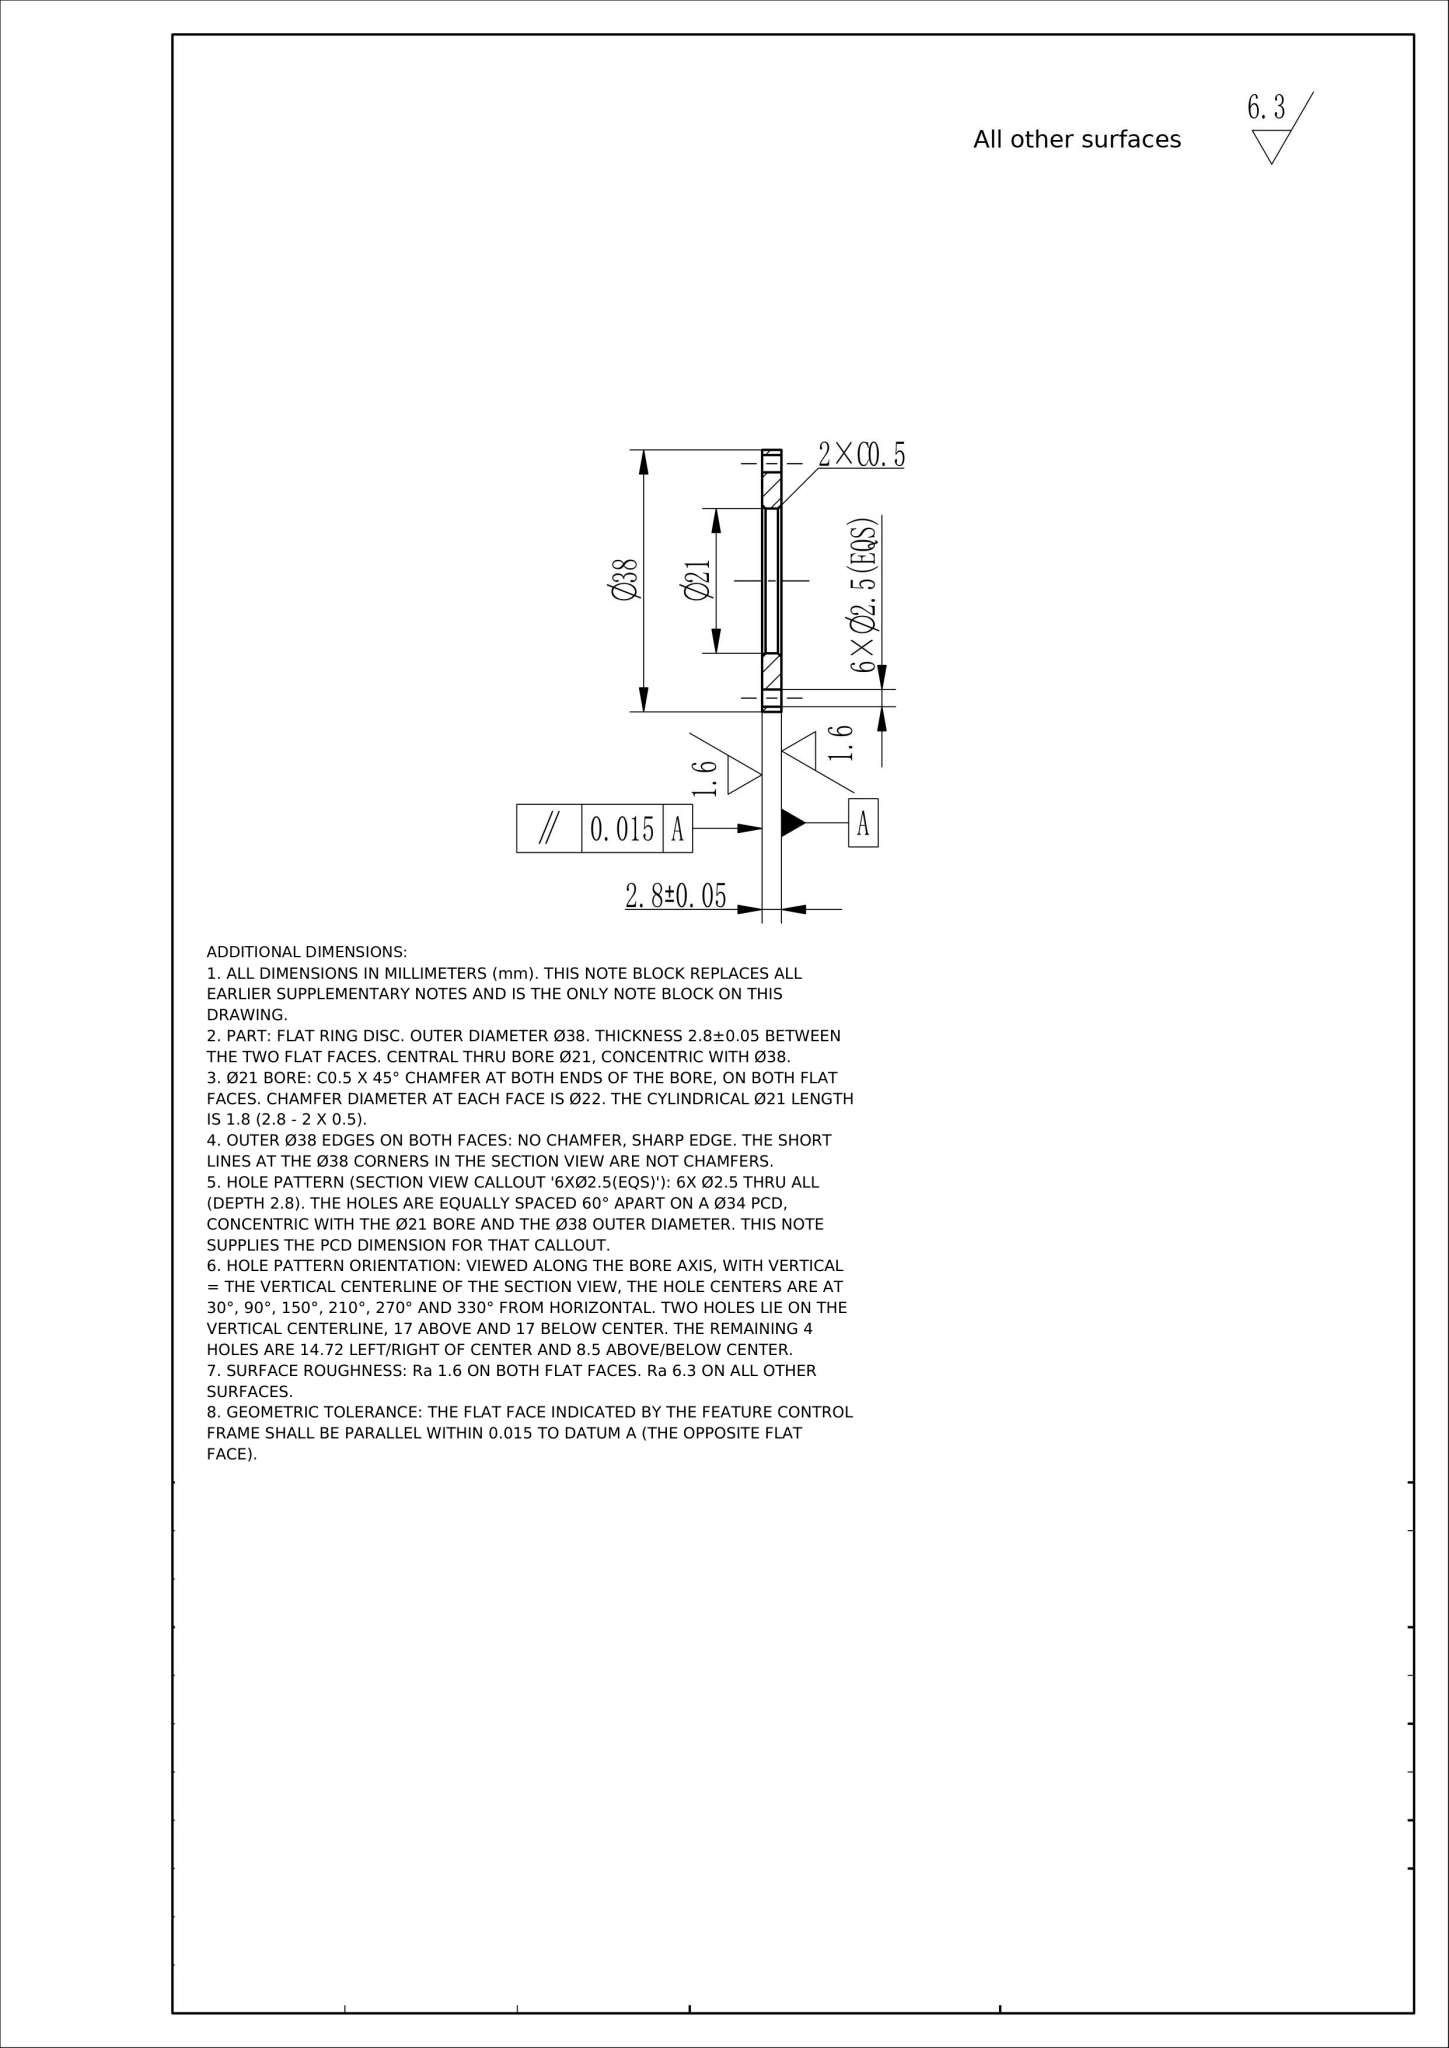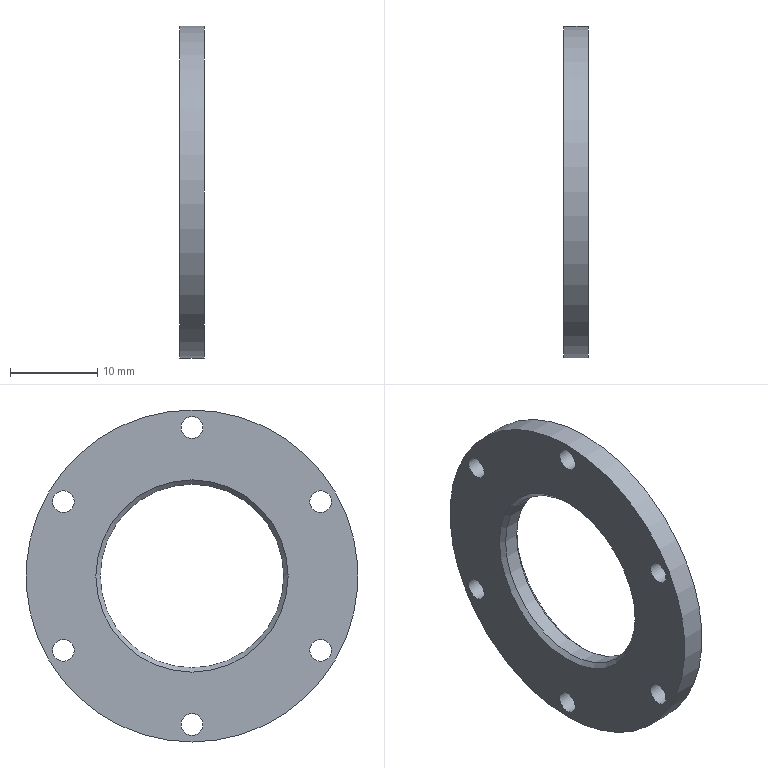Part | NX | mm | 1 solid | 12 faces | box 2.8 x 38 x 38 mm | volume 2106 mm3 | cylinder 8 | plane 2 | cone 2 | commonest cylinder face diameters 2.5 x6 38 x1 21 x1
STEP:
#1=CARTESIAN_POINT('',(0.,0.,0.));
#2=DIRECTION('',(0.,0.,1.));
#3=DIRECTION('',(1.,0.,0.));
#4=AXIS2_PLACEMENT_3D('',#1,#2,#3);
#5=(LENGTH_UNIT()NAMED_UNIT(*)SI_UNIT(.MILLI.,.METRE.));
#6=UNCERTAINTY_MEASURE_WITH_UNIT(LENGTH_MEASURE(0.00002),#5,'','');
#7=(NAMED_UNIT(*)PLANE_ANGLE_UNIT()SI_UNIT($,.RADIAN.));
#8=PLANE_ANGLE_MEASURE_WITH_UNIT(PLANE_ANGLE_MEASURE(0.01745),#7);
#9=DIMENSIONAL_EXPONENTS(0.,0.,0.,0.,0.,0.,0.);
#10=(CONVERSION_BASED_UNIT('',#8)NAMED_UNIT(#9)PLANE_ANGLE_UNIT());
#11=(NAMED_UNIT(*)SI_UNIT($,.STERADIAN.)SOLID_ANGLE_UNIT());
#12=(GEOMETRIC_REPRESENTATION_CONTEXT(3)GLOBAL_UNCERTAINTY_ASSIGNED_CONTEXT((#6))GLOBAL_UNIT_ASSIGNED_CONTEXT((#5,#10,#11))REPRESENTATION_CONTEXT('',''));
#13=SHAPE_REPRESENTATION('',(#4),#12);
#14=CARTESIAN_POINT('',(2.8,0.,-11.));
#15=VERTEX_POINT('',#14);
#16=CARTESIAN_POINT('',(2.8,0.,0.));
#17=DIRECTION('',(-1.,0.,0.));
#18=DIRECTION('',(0.,0.,-1.));
#19=AXIS2_PLACEMENT_3D('',#16,#17,#18);
#20=CIRCLE('',#19,11.);
#21=EDGE_CURVE('',#15,#15,#20,.T.);
#22=ORIENTED_EDGE('',*,*,#21,.T.);
#23=EDGE_LOOP('',(#22));
#24=FACE_BOUND('',#23,.T.);
#25=CARTESIAN_POINT('',(2.8,14.722,9.75));
#26=VERTEX_POINT('',#25);
#27=CARTESIAN_POINT('',(2.8,14.722,8.5));
#28=DIRECTION('',(-1.,0.,0.));
#29=DIRECTION('',(0.,0.,1.));
#30=AXIS2_PLACEMENT_3D('',#27,#28,#29);
#31=CIRCLE('',#30,1.25);
#32=EDGE_CURVE('',#26,#26,#31,.T.);
#33=ORIENTED_EDGE('',*,*,#32,.T.);
#34=EDGE_LOOP('',(#33));
#35=FACE_BOUND('',#34,.T.);
#36=CARTESIAN_POINT('',(2.8,14.722,-7.25));
#37=VERTEX_POINT('',#36);
#38=CARTESIAN_POINT('',(2.8,14.722,-8.5));
#39=DIRECTION('',(-1.,0.,0.));
#40=DIRECTION('',(0.,0.,1.));
#41=AXIS2_PLACEMENT_3D('',#38,#39,#40);
#42=CIRCLE('',#41,1.25);
#43=EDGE_CURVE('',#37,#37,#42,.T.);
#44=ORIENTED_EDGE('',*,*,#43,.T.);
#45=EDGE_LOOP('',(#44));
#46=FACE_BOUND('',#45,.T.);
#47=CARTESIAN_POINT('',(2.8,0.,-15.75));
#48=VERTEX_POINT('',#47);
#49=CARTESIAN_POINT('',(2.8,0.,-17.));
#50=DIRECTION('',(-1.,0.,0.));
#51=DIRECTION('',(0.,0.,1.));
#52=AXIS2_PLACEMENT_3D('',#49,#50,#51);
#53=CIRCLE('',#52,1.25);
#54=EDGE_CURVE('',#48,#48,#53,.T.);
#55=ORIENTED_EDGE('',*,*,#54,.T.);
#56=EDGE_LOOP('',(#55));
#57=FACE_BOUND('',#56,.T.);
#58=CARTESIAN_POINT('',(2.8,-14.722,-7.25));
#59=VERTEX_POINT('',#58);
#60=CARTESIAN_POINT('',(2.8,-14.722,-8.5));
#61=DIRECTION('',(-1.,0.,0.));
#62=DIRECTION('',(0.,0.,1.));
#63=AXIS2_PLACEMENT_3D('',#60,#61,#62);
#64=CIRCLE('',#63,1.25);
#65=EDGE_CURVE('',#59,#59,#64,.T.);
#66=ORIENTED_EDGE('',*,*,#65,.T.);
#67=EDGE_LOOP('',(#66));
#68=FACE_BOUND('',#67,.T.);
#69=CARTESIAN_POINT('',(2.8,-14.722,9.75));
#70=VERTEX_POINT('',#69);
#71=CARTESIAN_POINT('',(2.8,-14.722,8.5));
#72=DIRECTION('',(-1.,0.,0.));
#73=DIRECTION('',(0.,0.,1.));
#74=AXIS2_PLACEMENT_3D('',#71,#72,#73);
#75=CIRCLE('',#74,1.25);
#76=EDGE_CURVE('',#70,#70,#75,.T.);
#77=ORIENTED_EDGE('',*,*,#76,.T.);
#78=EDGE_LOOP('',(#77));
#79=FACE_BOUND('',#78,.T.);
#80=CARTESIAN_POINT('',(2.8,0.,18.25));
#81=VERTEX_POINT('',#80);
#82=CARTESIAN_POINT('',(2.8,0.,17.));
#83=DIRECTION('',(-1.,0.,0.));
#84=DIRECTION('',(0.,0.,1.));
#85=AXIS2_PLACEMENT_3D('',#82,#83,#84);
#86=CIRCLE('',#85,1.25);
#87=EDGE_CURVE('',#81,#81,#86,.T.);
#88=ORIENTED_EDGE('',*,*,#87,.T.);
#89=EDGE_LOOP('',(#88));
#90=FACE_BOUND('',#89,.T.);
#91=CARTESIAN_POINT('',(2.8,0.,-19.));
#92=VERTEX_POINT('',#91);
#93=CARTESIAN_POINT('',(2.8,0.,0.));
#94=DIRECTION('',(-1.,0.,0.));
#95=DIRECTION('',(0.,0.,-1.));
#96=AXIS2_PLACEMENT_3D('',#93,#94,#95);
#97=CIRCLE('',#96,19.);
#98=EDGE_CURVE('',#92,#92,#97,.T.);
#99=ORIENTED_EDGE('',*,*,#98,.F.);
#100=EDGE_LOOP('',(#99));
#101=FACE_BOUND('',#100,.T.);
#102=CARTESIAN_POINT('',(2.8,0.,0.));
#103=DIRECTION('',(1.,0.,0.));
#104=DIRECTION('',(0.,0.,-1.));
#105=AXIS2_PLACEMENT_3D('',#102,#103,#104);
#106=PLANE('',#105);
#107=ADVANCED_FACE('',(#24,#35,#46,#57,#68,#79,#90,#101),#106,.T.);
#108=CARTESIAN_POINT('',(0.,0.,11.));
#109=VERTEX_POINT('',#108);
#110=CARTESIAN_POINT('',(0.,0.,0.));
#111=DIRECTION('',(1.,0.,0.));
#112=DIRECTION('',(0.,0.,1.));
#113=AXIS2_PLACEMENT_3D('',#110,#111,#112);
#114=CIRCLE('',#113,11.);
#115=EDGE_CURVE('',#109,#109,#114,.T.);
#116=ORIENTED_EDGE('',*,*,#115,.T.);
#117=EDGE_LOOP('',(#116));
#118=FACE_BOUND('',#117,.T.);
#119=CARTESIAN_POINT('',(0.,14.722,9.75));
#120=VERTEX_POINT('',#119);
#121=CARTESIAN_POINT('',(0.,14.722,8.5));
#122=DIRECTION('',(-1.,0.,0.));
#123=DIRECTION('',(0.,0.,1.));
#124=AXIS2_PLACEMENT_3D('',#121,#122,#123);
#125=CIRCLE('',#124,1.25);
#126=EDGE_CURVE('',#120,#120,#125,.T.);
#127=ORIENTED_EDGE('',*,*,#126,.F.);
#128=EDGE_LOOP('',(#127));
#129=FACE_BOUND('',#128,.T.);
#130=CARTESIAN_POINT('',(0.,14.722,-7.25));
#131=VERTEX_POINT('',#130);
#132=CARTESIAN_POINT('',(0.,14.722,-8.5));
#133=DIRECTION('',(-1.,0.,0.));
#134=DIRECTION('',(0.,0.,1.));
#135=AXIS2_PLACEMENT_3D('',#132,#133,#134);
#136=CIRCLE('',#135,1.25);
#137=EDGE_CURVE('',#131,#131,#136,.T.);
#138=ORIENTED_EDGE('',*,*,#137,.F.);
#139=EDGE_LOOP('',(#138));
#140=FACE_BOUND('',#139,.T.);
#141=CARTESIAN_POINT('',(0.,0.,-15.75));
#142=VERTEX_POINT('',#141);
#143=CARTESIAN_POINT('',(0.,0.,-17.));
#144=DIRECTION('',(-1.,0.,0.));
#145=DIRECTION('',(0.,0.,1.));
#146=AXIS2_PLACEMENT_3D('',#143,#144,#145);
#147=CIRCLE('',#146,1.25);
#148=EDGE_CURVE('',#142,#142,#147,.T.);
#149=ORIENTED_EDGE('',*,*,#148,.F.);
#150=EDGE_LOOP('',(#149));
#151=FACE_BOUND('',#150,.T.);
#152=CARTESIAN_POINT('',(0.,-14.722,-7.25));
#153=VERTEX_POINT('',#152);
#154=CARTESIAN_POINT('',(0.,-14.722,-8.5));
#155=DIRECTION('',(-1.,0.,0.));
#156=DIRECTION('',(0.,0.,1.));
#157=AXIS2_PLACEMENT_3D('',#154,#155,#156);
#158=CIRCLE('',#157,1.25);
#159=EDGE_CURVE('',#153,#153,#158,.T.);
#160=ORIENTED_EDGE('',*,*,#159,.F.);
#161=EDGE_LOOP('',(#160));
#162=FACE_BOUND('',#161,.T.);
#163=CARTESIAN_POINT('',(0.,-14.722,9.75));
#164=VERTEX_POINT('',#163);
#165=CARTESIAN_POINT('',(0.,-14.722,8.5));
#166=DIRECTION('',(-1.,0.,0.));
#167=DIRECTION('',(0.,0.,1.));
#168=AXIS2_PLACEMENT_3D('',#165,#166,#167);
#169=CIRCLE('',#168,1.25);
#170=EDGE_CURVE('',#164,#164,#169,.T.);
#171=ORIENTED_EDGE('',*,*,#170,.F.);
#172=EDGE_LOOP('',(#171));
#173=FACE_BOUND('',#172,.T.);
#174=CARTESIAN_POINT('',(0.,0.,18.25));
#175=VERTEX_POINT('',#174);
#176=CARTESIAN_POINT('',(0.,0.,17.));
#177=DIRECTION('',(-1.,0.,0.));
#178=DIRECTION('',(0.,0.,1.));
#179=AXIS2_PLACEMENT_3D('',#176,#177,#178);
#180=CIRCLE('',#179,1.25);
#181=EDGE_CURVE('',#175,#175,#180,.T.);
#182=ORIENTED_EDGE('',*,*,#181,.F.);
#183=EDGE_LOOP('',(#182));
#184=FACE_BOUND('',#183,.T.);
#185=CARTESIAN_POINT('',(0.,0.,-19.));
#186=VERTEX_POINT('',#185);
#187=CARTESIAN_POINT('',(0.,0.,0.));
#188=DIRECTION('',(1.,0.,0.));
#189=DIRECTION('',(0.,0.,-1.));
#190=AXIS2_PLACEMENT_3D('',#187,#188,#189);
#191=CIRCLE('',#190,19.);
#192=EDGE_CURVE('',#186,#186,#191,.T.);
#193=ORIENTED_EDGE('',*,*,#192,.F.);
#194=EDGE_LOOP('',(#193));
#195=FACE_BOUND('',#194,.T.);
#196=CARTESIAN_POINT('',(0.,0.,0.));
#197=DIRECTION('',(-1.,0.,0.));
#198=DIRECTION('',(0.,0.,1.));
#199=AXIS2_PLACEMENT_3D('',#196,#197,#198);
#200=PLANE('',#199);
#201=ADVANCED_FACE('',(#118,#129,#140,#151,#162,#173,#184,#195),#200,.T.);
#202=ORIENTED_EDGE('',*,*,#98,.T.);
#203=EDGE_LOOP('',(#202));
#204=FACE_BOUND('',#203,.T.);
#205=ORIENTED_EDGE('',*,*,#192,.T.);
#206=EDGE_LOOP('',(#205));
#207=FACE_BOUND('',#206,.T.);
#208=CARTESIAN_POINT('',(0.,0.,0.));
#209=DIRECTION('',(1.,0.,0.));
#210=DIRECTION('',(0.,0.,-1.));
#211=AXIS2_PLACEMENT_3D('',#208,#209,#210);
#212=CYLINDRICAL_SURFACE('',#211,19.);
#213=ADVANCED_FACE('',(#204,#207),#212,.T.);
#214=CARTESIAN_POINT('',(0.5,0.,10.5));
#215=VERTEX_POINT('',#214);
#216=CARTESIAN_POINT('',(0.5,0.,0.));
#217=DIRECTION('',(-1.,0.,0.));
#218=DIRECTION('',(0.,0.,1.));
#219=AXIS2_PLACEMENT_3D('',#216,#217,#218);
#220=CIRCLE('',#219,10.5);
#221=EDGE_CURVE('',#215,#215,#220,.T.);
#222=ORIENTED_EDGE('',*,*,#221,.T.);
#223=EDGE_LOOP('',(#222));
#224=FACE_BOUND('',#223,.T.);
#225=CARTESIAN_POINT('',(2.3,0.,-10.5));
#226=VERTEX_POINT('',#225);
#227=CARTESIAN_POINT('',(2.3,0.,0.));
#228=DIRECTION('',(1.,0.,0.));
#229=DIRECTION('',(0.,0.,-1.));
#230=AXIS2_PLACEMENT_3D('',#227,#228,#229);
#231=CIRCLE('',#230,10.5);
#232=EDGE_CURVE('',#226,#226,#231,.T.);
#233=ORIENTED_EDGE('',*,*,#232,.T.);
#234=EDGE_LOOP('',(#233));
#235=FACE_BOUND('',#234,.T.);
#236=CARTESIAN_POINT('',(2.8,0.,0.));
#237=DIRECTION('',(-1.,0.,0.));
#238=DIRECTION('',(0.,0.,1.));
#239=AXIS2_PLACEMENT_3D('',#236,#237,#238);
#240=CYLINDRICAL_SURFACE('',#239,10.5);
#241=ADVANCED_FACE('',(#224,#235),#240,.F.);
#242=ORIENTED_EDGE('',*,*,#181,.T.);
#243=EDGE_LOOP('',(#242));
#244=FACE_BOUND('',#243,.T.);
#245=ORIENTED_EDGE('',*,*,#87,.F.);
#246=EDGE_LOOP('',(#245));
#247=FACE_BOUND('',#246,.T.);
#248=CARTESIAN_POINT('',(2.8,0.,17.));
#249=DIRECTION('',(-1.,0.,0.));
#250=DIRECTION('',(0.,0.,1.));
#251=AXIS2_PLACEMENT_3D('',#248,#249,#250);
#252=CYLINDRICAL_SURFACE('',#251,1.25);
#253=ADVANCED_FACE('',(#244,#247),#252,.F.);
#254=ORIENTED_EDGE('',*,*,#170,.T.);
#255=EDGE_LOOP('',(#254));
#256=FACE_BOUND('',#255,.T.);
#257=ORIENTED_EDGE('',*,*,#76,.F.);
#258=EDGE_LOOP('',(#257));
#259=FACE_BOUND('',#258,.T.);
#260=CARTESIAN_POINT('',(2.8,-14.722,8.5));
#261=DIRECTION('',(-1.,0.,0.));
#262=DIRECTION('',(0.,0.,1.));
#263=AXIS2_PLACEMENT_3D('',#260,#261,#262);
#264=CYLINDRICAL_SURFACE('',#263,1.25);
#265=ADVANCED_FACE('',(#256,#259),#264,.F.);
#266=ORIENTED_EDGE('',*,*,#159,.T.);
#267=EDGE_LOOP('',(#266));
#268=FACE_BOUND('',#267,.T.);
#269=ORIENTED_EDGE('',*,*,#65,.F.);
#270=EDGE_LOOP('',(#269));
#271=FACE_BOUND('',#270,.T.);
#272=CARTESIAN_POINT('',(2.8,-14.722,-8.5));
#273=DIRECTION('',(-1.,0.,0.));
#274=DIRECTION('',(0.,0.,1.));
#275=AXIS2_PLACEMENT_3D('',#272,#273,#274);
#276=CYLINDRICAL_SURFACE('',#275,1.25);
#277=ADVANCED_FACE('',(#268,#271),#276,.F.);
#278=ORIENTED_EDGE('',*,*,#148,.T.);
#279=EDGE_LOOP('',(#278));
#280=FACE_BOUND('',#279,.T.);
#281=ORIENTED_EDGE('',*,*,#54,.F.);
#282=EDGE_LOOP('',(#281));
#283=FACE_BOUND('',#282,.T.);
#284=CARTESIAN_POINT('',(2.8,0.,-17.));
#285=DIRECTION('',(-1.,0.,0.));
#286=DIRECTION('',(0.,0.,1.));
#287=AXIS2_PLACEMENT_3D('',#284,#285,#286);
#288=CYLINDRICAL_SURFACE('',#287,1.25);
#289=ADVANCED_FACE('',(#280,#283),#288,.F.);
#290=ORIENTED_EDGE('',*,*,#137,.T.);
#291=EDGE_LOOP('',(#290));
#292=FACE_BOUND('',#291,.T.);
#293=ORIENTED_EDGE('',*,*,#43,.F.);
#294=EDGE_LOOP('',(#293));
#295=FACE_BOUND('',#294,.T.);
#296=CARTESIAN_POINT('',(2.8,14.722,-8.5));
#297=DIRECTION('',(-1.,0.,0.));
#298=DIRECTION('',(0.,0.,1.));
#299=AXIS2_PLACEMENT_3D('',#296,#297,#298);
#300=CYLINDRICAL_SURFACE('',#299,1.25);
#301=ADVANCED_FACE('',(#292,#295),#300,.F.);
#302=ORIENTED_EDGE('',*,*,#126,.T.);
#303=EDGE_LOOP('',(#302));
#304=FACE_BOUND('',#303,.T.);
#305=ORIENTED_EDGE('',*,*,#32,.F.);
#306=EDGE_LOOP('',(#305));
#307=FACE_BOUND('',#306,.T.);
#308=CARTESIAN_POINT('',(2.8,14.722,8.5));
#309=DIRECTION('',(-1.,0.,0.));
#310=DIRECTION('',(0.,0.,1.));
#311=AXIS2_PLACEMENT_3D('',#308,#309,#310);
#312=CYLINDRICAL_SURFACE('',#311,1.25);
#313=ADVANCED_FACE('',(#304,#307),#312,.F.);
#314=ORIENTED_EDGE('',*,*,#115,.F.);
#315=EDGE_LOOP('',(#314));
#316=FACE_BOUND('',#315,.T.);
#317=ORIENTED_EDGE('',*,*,#221,.F.);
#318=EDGE_LOOP('',(#317));
#319=FACE_BOUND('',#318,.T.);
#320=CARTESIAN_POINT('',(0.5,0.,0.));
#321=DIRECTION('',(-1.,0.,0.));
#322=DIRECTION('',(-0.,0.,1.));
#323=AXIS2_PLACEMENT_3D('',#320,#321,#322);
#324=CONICAL_SURFACE('',#323,10.5,45.);
#325=ADVANCED_FACE('',(#316,#319),#324,.F.);
#326=ORIENTED_EDGE('',*,*,#232,.F.);
#327=EDGE_LOOP('',(#326));
#328=FACE_BOUND('',#327,.T.);
#329=ORIENTED_EDGE('',*,*,#21,.F.);
#330=EDGE_LOOP('',(#329));
#331=FACE_BOUND('',#330,.T.);
#332=CARTESIAN_POINT('',(2.8,0.,0.));
#333=DIRECTION('',(1.,0.,0.));
#334=DIRECTION('',(-0.,0.,-1.));
#335=AXIS2_PLACEMENT_3D('',#332,#333,#334);
#336=CONICAL_SURFACE('',#335,11.,45.);
#337=ADVANCED_FACE('',(#328,#331),#336,.F.);
#338=CLOSED_SHELL('',(#107,#201,#213,#241,#253,#265,#277,#289,#301,#313,#325,#337));
#339=MANIFOLD_SOLID_BREP('',#338);
#340=ADVANCED_BREP_SHAPE_REPRESENTATION('',(#339),#12);
#341=SHAPE_REPRESENTATION_RELATIONSHIP('','',#13,#340);
#342=PRESENTATION_LAYER_ASSIGNMENT('','',(#339));
#343=COLOUR_RGB('',0.8,0.6,0.);
#344=FILL_AREA_STYLE_COLOUR('',#343);
#345=FILL_AREA_STYLE('',(#344));
#346=SURFACE_STYLE_FILL_AREA(#345);
#347=SURFACE_SIDE_STYLE('',(#346));
#348=SURFACE_STYLE_USAGE(.BOTH.,#347);
#349=PRESENTATION_STYLE_ASSIGNMENT((#348));
#350=STYLED_ITEM('',(#349),#339);
#351=MECHANICAL_DESIGN_GEOMETRIC_PRESENTATION_REPRESENTATION('',(#350),#12);